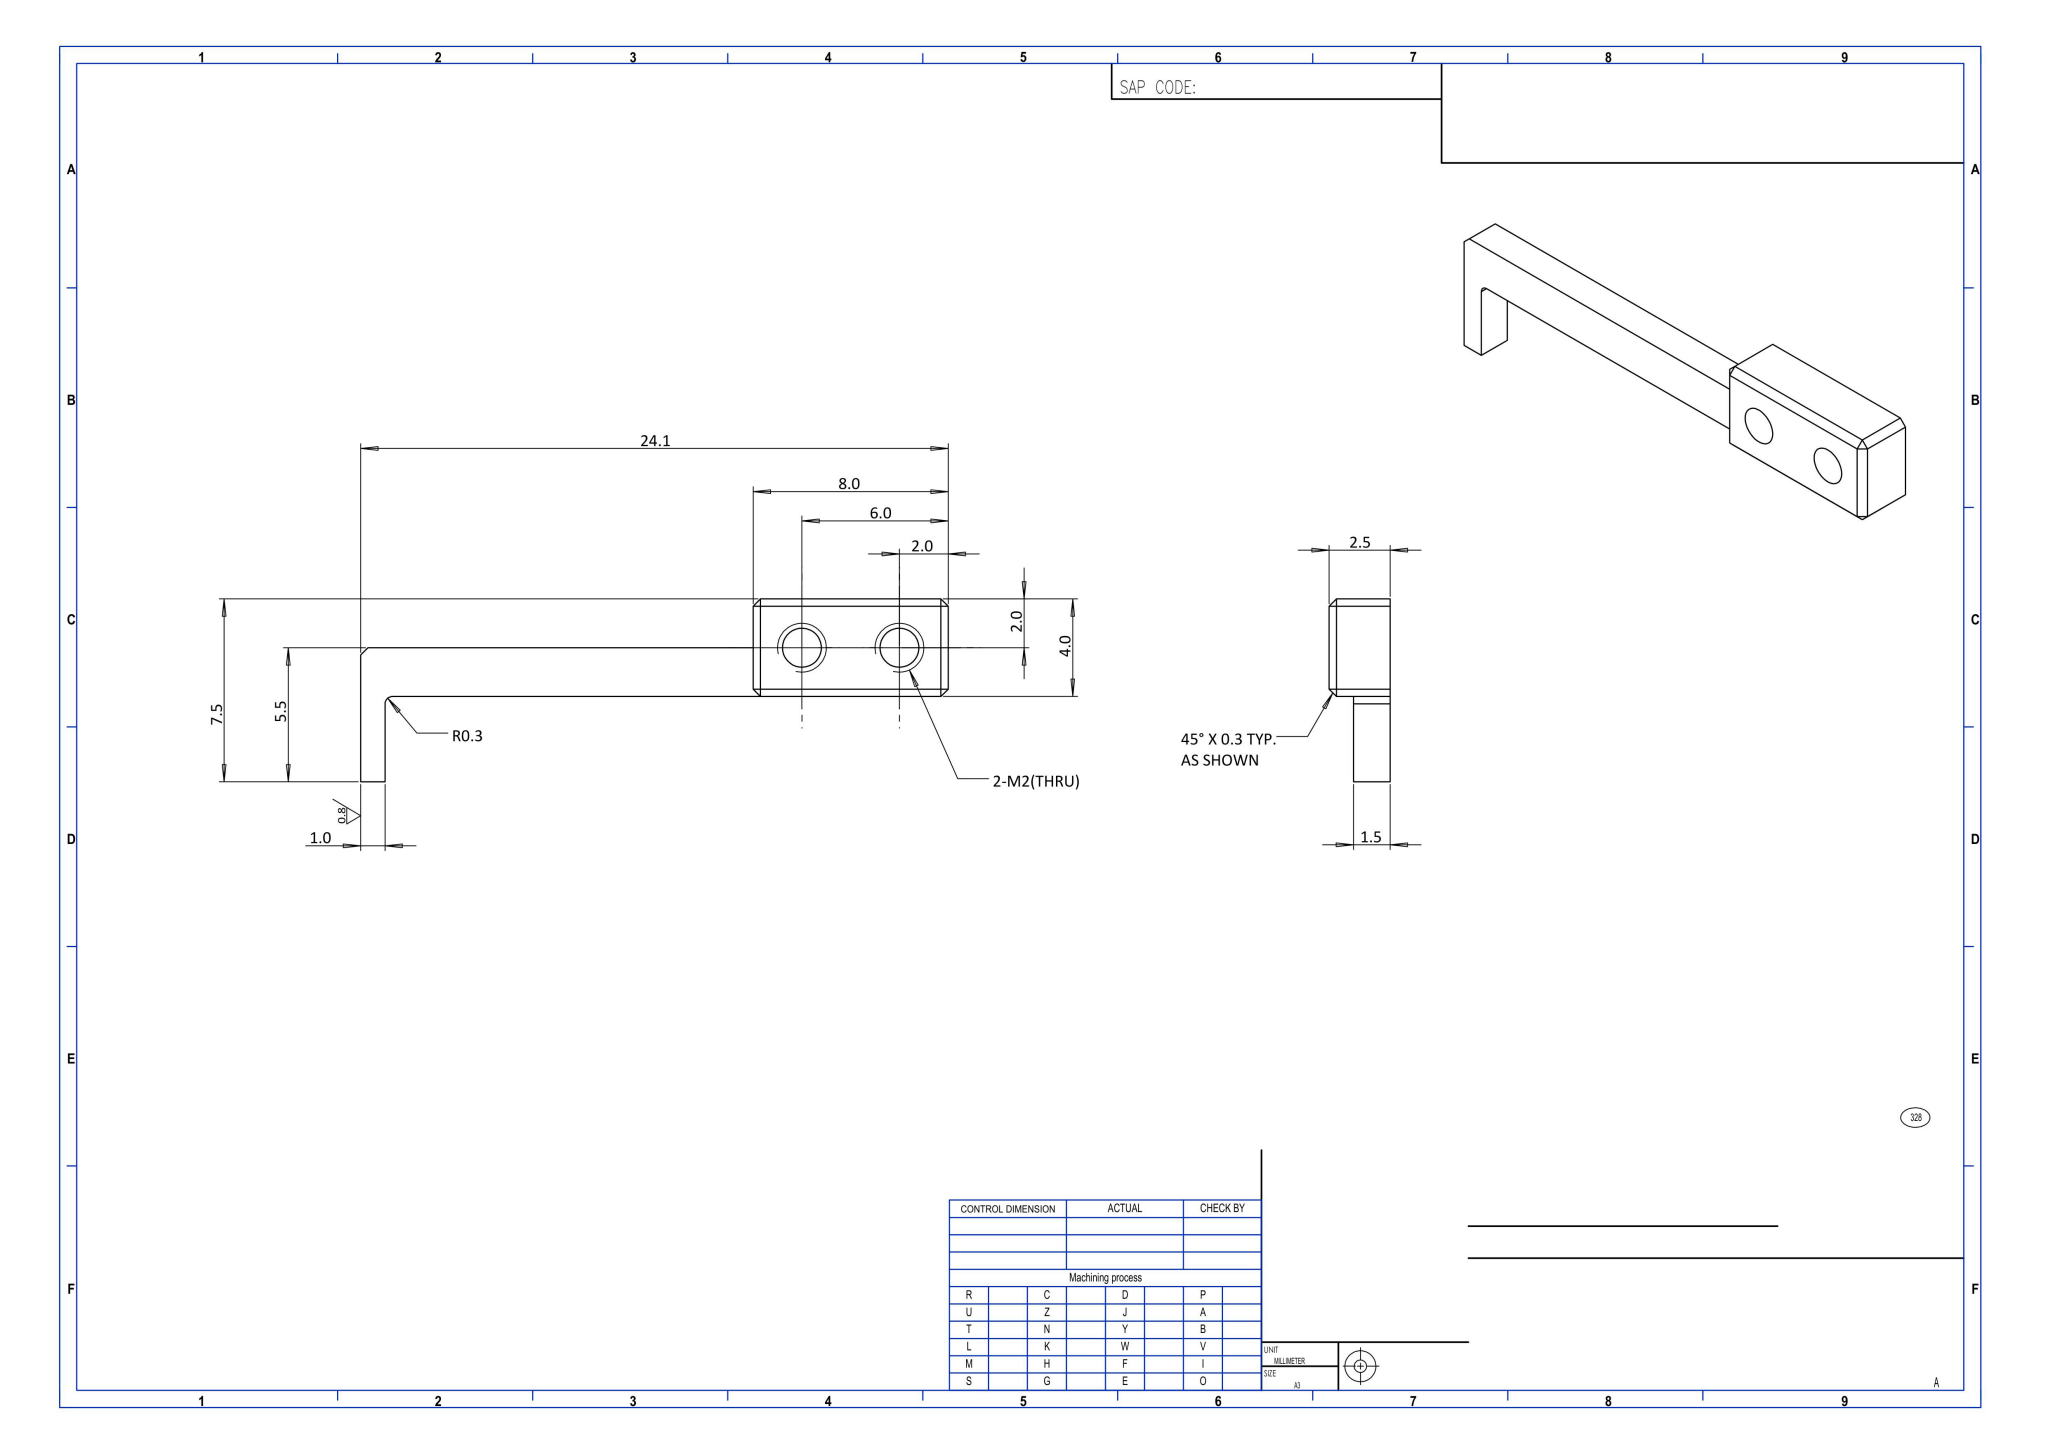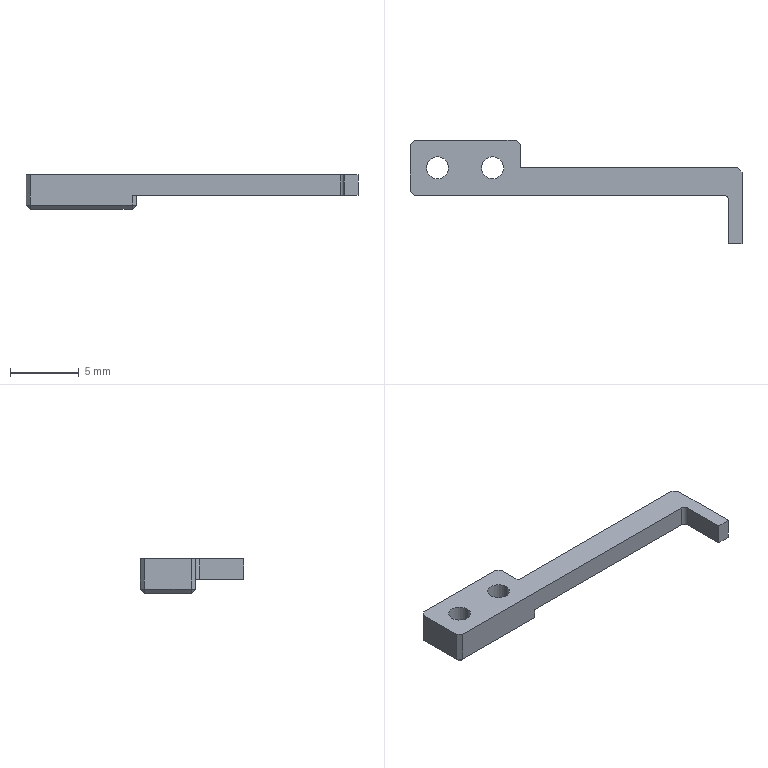Part | NX | mm | 1 solid | 29 faces | box 24.1 x 7.5 x 2.5 mm | volume 122 mm3 | plane 24 | cylinder 5 | commonest cylinder face diameters 1.6 x4 0.6 x1
STEP:
#1=COLOUR_RGB('',0.7529,0.7529,0.7529);
#2=FILL_AREA_STYLE_COLOUR('',#1);
#3=FILL_AREA_STYLE('',(#2));
#4=SURFACE_STYLE_FILL_AREA(#3);
#5=SURFACE_SIDE_STYLE('',(#4));
#6=SURFACE_STYLE_USAGE(.BOTH.,#5);
#7=PRESENTATION_STYLE_ASSIGNMENT((#6));
#8=CARTESIAN_POINT('',(1.2,1.75,-2.5));
#9=VERTEX_POINT('',#8);
#10=CARTESIAN_POINT('',(1.2,1.75,0.));
#11=VERTEX_POINT('',#10);
#12=CARTESIAN_POINT('',(1.2,1.75,0.));
#13=DIRECTION('',(0.,0.,1.));
#14=VECTOR('',#13,1000.);
#15=LINE('',#12,#14);
#16=EDGE_CURVE('',#9,#11,#15,.T.);
#17=ORIENTED_EDGE('',*,*,#16,.F.);
#18=CARTESIAN_POINT('',(2.8,1.75,-2.5));
#19=VERTEX_POINT('',#18);
#20=CARTESIAN_POINT('',(2.,1.75,-2.5));
#21=DIRECTION('',(0.,0.,1.));
#22=DIRECTION('',(1.,0.,0.));
#23=AXIS2_PLACEMENT_3D('',#20,#21,#22);
#24=CIRCLE('',#23,0.8);
#25=EDGE_CURVE('',#19,#9,#24,.T.);
#26=ORIENTED_EDGE('',*,*,#25,.F.);
#27=CARTESIAN_POINT('',(2.8,1.75,0.));
#28=VERTEX_POINT('',#27);
#29=CARTESIAN_POINT('',(2.8,1.75,0.));
#30=DIRECTION('',(0.,0.,1.));
#31=VECTOR('',#30,1000.);
#32=LINE('',#29,#31);
#33=EDGE_CURVE('',#19,#28,#32,.T.);
#34=ORIENTED_EDGE('',*,*,#33,.T.);
#35=CARTESIAN_POINT('',(2.,1.75,0.));
#36=DIRECTION('',(0.,0.,1.));
#37=DIRECTION('',(1.,0.,0.));
#38=AXIS2_PLACEMENT_3D('',#35,#36,#37);
#39=CIRCLE('',#38,0.8);
#40=EDGE_CURVE('',#28,#11,#39,.T.);
#41=ORIENTED_EDGE('',*,*,#40,.T.);
#42=EDGE_LOOP('',(#17,#26,#34,#41));
#43=FACE_OUTER_BOUND('',#42,.T.);
#44=CARTESIAN_POINT('',(2.,1.75,0.));
#45=DIRECTION('',(0.,0.,1.));
#46=DIRECTION('',(1.,0.,0.));
#47=AXIS2_PLACEMENT_3D('',#44,#45,#46);
#48=CYLINDRICAL_SURFACE('',#47,0.8);
#49=ADVANCED_FACE('',(#43),#48,.F.);
#50=STYLED_ITEM('',(#7),#49);
#51=(LENGTH_UNIT()NAMED_UNIT(*)SI_UNIT(.MILLI.,.METRE.));
#52=UNCERTAINTY_MEASURE_WITH_UNIT(LENGTH_MEASURE(0.00001),#51,'','');
#53=(NAMED_UNIT(*)PLANE_ANGLE_UNIT()SI_UNIT($,.RADIAN.));
#54=(NAMED_UNIT(*)SI_UNIT($,.STERADIAN.)SOLID_ANGLE_UNIT());
#55=(GEOMETRIC_REPRESENTATION_CONTEXT(3)GLOBAL_UNCERTAINTY_ASSIGNED_CONTEXT((#52))GLOBAL_UNIT_ASSIGNED_CONTEXT((#51,#53,#54))REPRESENTATION_CONTEXT('',''));
#56=MECHANICAL_DESIGN_GEOMETRIC_PRESENTATION_REPRESENTATION('',(#50),#55);
#57=COLOUR_RGB('',0.7529,0.7529,0.7529);
#58=FILL_AREA_STYLE_COLOUR('',#57);
#59=FILL_AREA_STYLE('',(#58));
#60=SURFACE_STYLE_FILL_AREA(#59);
#61=SURFACE_SIDE_STYLE('',(#60));
#62=SURFACE_STYLE_USAGE(.BOTH.,#61);
#63=PRESENTATION_STYLE_ASSIGNMENT((#62));
#64=CARTESIAN_POINT('',(2.,1.75,-2.5));
#65=DIRECTION('',(0.,0.,1.));
#66=DIRECTION('',(1.,0.,0.));
#67=AXIS2_PLACEMENT_3D('',#64,#65,#66);
#68=CIRCLE('',#67,0.8);
#69=EDGE_CURVE('',#9,#19,#68,.T.);
#70=ORIENTED_EDGE('',*,*,#69,.F.);
#71=ORIENTED_EDGE('',*,*,#16,.T.);
#72=CARTESIAN_POINT('',(2.,1.75,0.));
#73=DIRECTION('',(0.,0.,1.));
#74=DIRECTION('',(1.,0.,0.));
#75=AXIS2_PLACEMENT_3D('',#72,#73,#74);
#76=CIRCLE('',#75,0.8);
#77=EDGE_CURVE('',#11,#28,#76,.T.);
#78=ORIENTED_EDGE('',*,*,#77,.T.);
#79=ORIENTED_EDGE('',*,*,#33,.F.);
#80=EDGE_LOOP('',(#70,#71,#78,#79));
#81=FACE_OUTER_BOUND('',#80,.T.);
#82=CARTESIAN_POINT('',(2.,1.75,0.));
#83=DIRECTION('',(0.,0.,1.));
#84=DIRECTION('',(1.,0.,0.));
#85=AXIS2_PLACEMENT_3D('',#82,#83,#84);
#86=CYLINDRICAL_SURFACE('',#85,0.8);
#87=ADVANCED_FACE('',(#81),#86,.F.);
#88=CARTESIAN_POINT('',(5.2,1.75,-2.5));
#89=VERTEX_POINT('',#88);
#90=CARTESIAN_POINT('',(6.8,1.75,-2.5));
#91=VERTEX_POINT('',#90);
#92=CARTESIAN_POINT('',(6.,1.75,-2.5));
#93=DIRECTION('',(0.,0.,1.));
#94=DIRECTION('',(1.,0.,0.));
#95=AXIS2_PLACEMENT_3D('',#92,#93,#94);
#96=CIRCLE('',#95,0.8);
#97=EDGE_CURVE('',#89,#91,#96,.T.);
#98=ORIENTED_EDGE('',*,*,#97,.F.);
#99=CARTESIAN_POINT('',(5.2,1.75,0.));
#100=VERTEX_POINT('',#99);
#101=CARTESIAN_POINT('',(5.2,1.75,0.));
#102=DIRECTION('',(0.,0.,1.));
#103=VECTOR('',#102,1000.);
#104=LINE('',#101,#103);
#105=EDGE_CURVE('',#89,#100,#104,.T.);
#106=ORIENTED_EDGE('',*,*,#105,.T.);
#107=CARTESIAN_POINT('',(6.8,1.75,0.));
#108=VERTEX_POINT('',#107);
#109=CARTESIAN_POINT('',(6.,1.75,0.));
#110=DIRECTION('',(0.,0.,1.));
#111=DIRECTION('',(1.,0.,0.));
#112=AXIS2_PLACEMENT_3D('',#109,#110,#111);
#113=CIRCLE('',#112,0.8);
#114=EDGE_CURVE('',#100,#108,#113,.T.);
#115=ORIENTED_EDGE('',*,*,#114,.T.);
#116=CARTESIAN_POINT('',(6.8,1.75,0.));
#117=DIRECTION('',(0.,0.,1.));
#118=VECTOR('',#117,1000.);
#119=LINE('',#116,#118);
#120=EDGE_CURVE('',#91,#108,#119,.T.);
#121=ORIENTED_EDGE('',*,*,#120,.F.);
#122=EDGE_LOOP('',(#98,#106,#115,#121));
#123=FACE_OUTER_BOUND('',#122,.T.);
#124=CARTESIAN_POINT('',(6.,1.75,0.));
#125=DIRECTION('',(0.,0.,1.));
#126=DIRECTION('',(1.,0.,0.));
#127=AXIS2_PLACEMENT_3D('',#124,#125,#126);
#128=CYLINDRICAL_SURFACE('',#127,0.8);
#129=ADVANCED_FACE('',(#123),#128,.F.);
#130=CARTESIAN_POINT('',(24.1,-3.75,-1.5));
#131=VERTEX_POINT('',#130);
#132=CARTESIAN_POINT('',(24.1,1.45,-1.5));
#133=VERTEX_POINT('',#132);
#134=CARTESIAN_POINT('',(24.1,-3.75,-1.5));
#135=DIRECTION('',(-0.,1.,0.));
#136=VECTOR('',#135,1000.);
#137=LINE('',#134,#136);
#138=EDGE_CURVE('',#131,#133,#137,.T.);
#139=ORIENTED_EDGE('',*,*,#138,.T.);
#140=CARTESIAN_POINT('',(24.1,1.45,0.));
#141=VERTEX_POINT('',#140);
#142=CARTESIAN_POINT('',(24.1,1.45,0.));
#143=DIRECTION('',(0.,0.,1.));
#144=VECTOR('',#143,1000.);
#145=LINE('',#142,#144);
#146=EDGE_CURVE('',#133,#141,#145,.T.);
#147=ORIENTED_EDGE('',*,*,#146,.T.);
#148=CARTESIAN_POINT('',(24.1,-3.75,0.));
#149=VERTEX_POINT('',#148);
#150=CARTESIAN_POINT('',(24.1,3.75,0.));
#151=DIRECTION('',(0.,1.,0.));
#152=VECTOR('',#151,1000.);
#153=LINE('',#150,#152);
#154=EDGE_CURVE('',#149,#141,#153,.T.);
#155=ORIENTED_EDGE('',*,*,#154,.F.);
#156=CARTESIAN_POINT('',(24.1,-3.75,-2.5));
#157=DIRECTION('',(0.,0.,1.));
#158=VECTOR('',#157,1000.);
#159=LINE('',#156,#158);
#160=EDGE_CURVE('',#131,#149,#159,.T.);
#161=ORIENTED_EDGE('',*,*,#160,.F.);
#162=EDGE_LOOP('',(#139,#147,#155,#161));
#163=FACE_OUTER_BOUND('',#162,.T.);
#164=CARTESIAN_POINT('',(24.1,3.75,-2.5));
#165=DIRECTION('',(1.,0.,0.));
#166=DIRECTION('',(0.,0.,-1.));
#167=AXIS2_PLACEMENT_3D('',#164,#165,#166);
#168=PLANE('',#167);
#169=ADVANCED_FACE('',(#163),#168,.T.);
#170=CARTESIAN_POINT('',(23.1,-3.75,-1.5));
#171=VERTEX_POINT('',#170);
#172=CARTESIAN_POINT('',(24.1,-3.75,-1.5));
#173=DIRECTION('',(1.,0.,-0.));
#174=VECTOR('',#173,1000.);
#175=LINE('',#172,#174);
#176=EDGE_CURVE('',#171,#131,#175,.T.);
#177=ORIENTED_EDGE('',*,*,#176,.T.);
#178=ORIENTED_EDGE('',*,*,#160,.T.);
#179=CARTESIAN_POINT('',(23.1,-3.75,0.));
#180=VERTEX_POINT('',#179);
#181=CARTESIAN_POINT('',(24.1,-3.75,0.));
#182=DIRECTION('',(1.,-0.,0.));
#183=VECTOR('',#182,1000.);
#184=LINE('',#181,#183);
#185=EDGE_CURVE('',#180,#149,#184,.T.);
#186=ORIENTED_EDGE('',*,*,#185,.F.);
#187=CARTESIAN_POINT('',(23.1,-3.75,-2.5));
#188=DIRECTION('',(0.,0.,1.));
#189=VECTOR('',#188,1000.);
#190=LINE('',#187,#189);
#191=EDGE_CURVE('',#171,#180,#190,.T.);
#192=ORIENTED_EDGE('',*,*,#191,.F.);
#193=EDGE_LOOP('',(#177,#178,#186,#192));
#194=FACE_OUTER_BOUND('',#193,.T.);
#195=CARTESIAN_POINT('',(24.1,-3.75,-2.5));
#196=DIRECTION('',(-0.,-1.,0.));
#197=DIRECTION('',(1.,-0.,0.));
#198=AXIS2_PLACEMENT_3D('',#195,#196,#197);
#199=PLANE('',#198);
#200=ADVANCED_FACE('',(#194),#199,.T.);
#201=CARTESIAN_POINT('',(-0.,3.45,0.));
#202=VERTEX_POINT('',#201);
#203=CARTESIAN_POINT('',(-0.,0.05,0.));
#204=VERTEX_POINT('',#203);
#205=CARTESIAN_POINT('',(-0.,3.75,0.));
#206=DIRECTION('',(0.,-1.,0.));
#207=VECTOR('',#206,1000.);
#208=LINE('',#205,#207);
#209=EDGE_CURVE('',#202,#204,#208,.T.);
#210=ORIENTED_EDGE('',*,*,#209,.F.);
#211=CARTESIAN_POINT('',(-0.,3.45,-2.2));
#212=VERTEX_POINT('',#211);
#213=CARTESIAN_POINT('',(-0.,3.45,-2.5));
#214=DIRECTION('',(0.,0.,-1.));
#215=VECTOR('',#214,1000.);
#216=LINE('',#213,#215);
#217=EDGE_CURVE('',#202,#212,#216,.T.);
#218=ORIENTED_EDGE('',*,*,#217,.T.);
#219=CARTESIAN_POINT('',(-0.,0.05,-2.2));
#220=VERTEX_POINT('',#219);
#221=CARTESIAN_POINT('',(-0.,3.75,-2.2));
#222=DIRECTION('',(0.,-1.,0.));
#223=VECTOR('',#222,1000.);
#224=LINE('',#221,#223);
#225=EDGE_CURVE('',#212,#220,#224,.T.);
#226=ORIENTED_EDGE('',*,*,#225,.T.);
#227=CARTESIAN_POINT('',(-0.,0.05,0.));
#228=DIRECTION('',(0.,0.,1.));
#229=VECTOR('',#228,1000.);
#230=LINE('',#227,#229);
#231=EDGE_CURVE('',#220,#204,#230,.T.);
#232=ORIENTED_EDGE('',*,*,#231,.T.);
#233=EDGE_LOOP('',(#210,#218,#226,#232));
#234=FACE_OUTER_BOUND('',#233,.T.);
#235=CARTESIAN_POINT('',(-0.,3.75,-2.5));
#236=DIRECTION('',(-1.,0.,0.));
#237=DIRECTION('',(0.,0.,1.));
#238=AXIS2_PLACEMENT_3D('',#235,#236,#237);
#239=PLANE('',#238);
#240=ADVANCED_FACE('',(#234),#239,.T.);
#241=CARTESIAN_POINT('',(7.7,3.75,-2.2));
#242=VERTEX_POINT('',#241);
#243=CARTESIAN_POINT('',(0.3,3.75,-2.2));
#244=VERTEX_POINT('',#243);
#245=CARTESIAN_POINT('',(24.1,3.75,-2.2));
#246=DIRECTION('',(-1.,-0.,0.));
#247=VECTOR('',#246,1000.);
#248=LINE('',#245,#247);
#249=EDGE_CURVE('',#242,#244,#248,.T.);
#250=ORIENTED_EDGE('',*,*,#249,.T.);
#251=CARTESIAN_POINT('',(0.3,3.75,0.));
#252=VERTEX_POINT('',#251);
#253=CARTESIAN_POINT('',(0.3,3.75,-2.5));
#254=DIRECTION('',(0.,0.,1.));
#255=VECTOR('',#254,1000.);
#256=LINE('',#253,#255);
#257=EDGE_CURVE('',#244,#252,#256,.T.);
#258=ORIENTED_EDGE('',*,*,#257,.T.);
#259=CARTESIAN_POINT('',(7.7,3.75,0.));
#260=VERTEX_POINT('',#259);
#261=CARTESIAN_POINT('',(24.1,3.75,0.));
#262=DIRECTION('',(-1.,-0.,0.));
#263=VECTOR('',#262,1000.);
#264=LINE('',#261,#263);
#265=EDGE_CURVE('',#260,#252,#264,.T.);
#266=ORIENTED_EDGE('',*,*,#265,.F.);
#267=CARTESIAN_POINT('',(7.7,3.75,-2.5));
#268=DIRECTION('',(-0.,-0.,-1.));
#269=VECTOR('',#268,1000.);
#270=LINE('',#267,#269);
#271=EDGE_CURVE('',#260,#242,#270,.T.);
#272=ORIENTED_EDGE('',*,*,#271,.T.);
#273=EDGE_LOOP('',(#250,#258,#266,#272));
#274=FACE_OUTER_BOUND('',#273,.T.);
#275=CARTESIAN_POINT('',(24.1,3.75,-2.5));
#276=DIRECTION('',(-0.,1.,0.));
#277=DIRECTION('',(-1.,-0.,0.));
#278=AXIS2_PLACEMENT_3D('',#275,#276,#277);
#279=PLANE('',#278);
#280=ADVANCED_FACE('',(#274),#279,.T.);
#281=CARTESIAN_POINT('',(0.3,0.05,-2.5));
#282=VERTEX_POINT('',#281);
#283=CARTESIAN_POINT('',(0.3,3.45,-2.5));
#284=VERTEX_POINT('',#283);
#285=CARTESIAN_POINT('',(0.3,0.,-2.5));
#286=DIRECTION('',(0.,1.,0.));
#287=VECTOR('',#286,1000.);
#288=LINE('',#285,#287);
#289=EDGE_CURVE('',#282,#284,#288,.T.);
#290=ORIENTED_EDGE('',*,*,#289,.T.);
#291=CARTESIAN_POINT('',(7.7,3.45,-2.5));
#292=VERTEX_POINT('',#291);
#293=CARTESIAN_POINT('',(-0.,3.45,-2.5));
#294=DIRECTION('',(1.,0.,0.));
#295=VECTOR('',#294,1000.);
#296=LINE('',#293,#295);
#297=EDGE_CURVE('',#284,#292,#296,.T.);
#298=ORIENTED_EDGE('',*,*,#297,.T.);
#299=CARTESIAN_POINT('',(7.7,0.05,-2.5));
#300=VERTEX_POINT('',#299);
#301=CARTESIAN_POINT('',(7.7,-0.25,-2.5));
#302=DIRECTION('',(0.,-1.,0.));
#303=VECTOR('',#302,1000.);
#304=LINE('',#301,#303);
#305=EDGE_CURVE('',#292,#300,#304,.T.);
#306=ORIENTED_EDGE('',*,*,#305,.T.);
#307=CARTESIAN_POINT('',(-0.,0.05,-2.5));
#308=DIRECTION('',(-1.,-0.,0.));
#309=VECTOR('',#308,1000.);
#310=LINE('',#307,#309);
#311=EDGE_CURVE('',#300,#282,#310,.T.);
#312=ORIENTED_EDGE('',*,*,#311,.T.);
#313=EDGE_LOOP('',(#290,#298,#306,#312));
#314=FACE_OUTER_BOUND('',#313,.T.);
#315=ORIENTED_EDGE('',*,*,#25,.T.);
#316=ORIENTED_EDGE('',*,*,#69,.T.);
#317=EDGE_LOOP('',(#315,#316));
#318=FACE_BOUND('',#317,.T.);
#319=CARTESIAN_POINT('',(6.,1.75,-2.5));
#320=DIRECTION('',(0.,0.,1.));
#321=DIRECTION('',(1.,0.,0.));
#322=AXIS2_PLACEMENT_3D('',#319,#320,#321);
#323=CIRCLE('',#322,0.8);
#324=EDGE_CURVE('',#91,#89,#323,.T.);
#325=ORIENTED_EDGE('',*,*,#324,.T.);
#326=ORIENTED_EDGE('',*,*,#97,.T.);
#327=EDGE_LOOP('',(#325,#326));
#328=FACE_BOUND('',#327,.T.);
#329=CARTESIAN_POINT('',(0.,0.,-2.5));
#330=DIRECTION('',(0.,0.,-1.));
#331=DIRECTION('',(-1.,0.,0.));
#332=AXIS2_PLACEMENT_3D('',#329,#330,#331);
#333=PLANE('',#332);
#334=ADVANCED_FACE('',(#314,#318,#328),#333,.T.);
#335=ORIENTED_EDGE('',*,*,#40,.F.);
#336=ORIENTED_EDGE('',*,*,#77,.F.);
#337=EDGE_LOOP('',(#335,#336));
#338=FACE_BOUND('',#337,.T.);
#339=CARTESIAN_POINT('',(6.,1.75,0.));
#340=DIRECTION('',(0.,0.,1.));
#341=DIRECTION('',(1.,0.,0.));
#342=AXIS2_PLACEMENT_3D('',#339,#340,#341);
#343=CIRCLE('',#342,0.8);
#344=EDGE_CURVE('',#108,#100,#343,.T.);
#345=ORIENTED_EDGE('',*,*,#344,.F.);
#346=ORIENTED_EDGE('',*,*,#114,.F.);
#347=EDGE_LOOP('',(#345,#346));
#348=FACE_BOUND('',#347,.T.);
#349=ORIENTED_EDGE('',*,*,#154,.T.);
#350=CARTESIAN_POINT('',(23.8,1.75,0.));
#351=VERTEX_POINT('',#350);
#352=CARTESIAN_POINT('',(24.1,1.45,0.));
#353=DIRECTION('',(-0.7071,0.7071,0.));
#354=VECTOR('',#353,1000.);
#355=LINE('',#352,#354);
#356=EDGE_CURVE('',#141,#351,#355,.T.);
#357=ORIENTED_EDGE('',*,*,#356,.T.);
#358=CARTESIAN_POINT('',(8.,1.75,0.));
#359=VERTEX_POINT('',#358);
#360=CARTESIAN_POINT('',(24.1,1.75,0.));
#361=DIRECTION('',(1.,0.,0.));
#362=VECTOR('',#361,1000.);
#363=LINE('',#360,#362);
#364=EDGE_CURVE('',#359,#351,#363,.T.);
#365=ORIENTED_EDGE('',*,*,#364,.F.);
#366=CARTESIAN_POINT('',(8.,3.45,0.));
#367=VERTEX_POINT('',#366);
#368=CARTESIAN_POINT('',(8.,3.75,0.));
#369=DIRECTION('',(0.,-1.,0.));
#370=VECTOR('',#369,1000.);
#371=LINE('',#368,#370);
#372=EDGE_CURVE('',#367,#359,#371,.T.);
#373=ORIENTED_EDGE('',*,*,#372,.F.);
#374=CARTESIAN_POINT('',(8.,3.45,0.));
#375=DIRECTION('',(-0.7071,0.7071,0.));
#376=VECTOR('',#375,1000.);
#377=LINE('',#374,#376);
#378=EDGE_CURVE('',#367,#260,#377,.T.);
#379=ORIENTED_EDGE('',*,*,#378,.T.);
#380=ORIENTED_EDGE('',*,*,#265,.T.);
#381=CARTESIAN_POINT('',(0.3,3.75,0.));
#382=DIRECTION('',(-0.7071,-0.7071,0.));
#383=VECTOR('',#382,1000.);
#384=LINE('',#381,#383);
#385=EDGE_CURVE('',#252,#202,#384,.T.);
#386=ORIENTED_EDGE('',*,*,#385,.T.);
#387=ORIENTED_EDGE('',*,*,#209,.T.);
#388=CARTESIAN_POINT('',(0.3,-0.25,0.));
#389=VERTEX_POINT('',#388);
#390=CARTESIAN_POINT('',(-0.,0.05,0.));
#391=DIRECTION('',(0.7071,-0.7071,0.));
#392=VECTOR('',#391,1000.);
#393=LINE('',#390,#392);
#394=EDGE_CURVE('',#204,#389,#393,.T.);
#395=ORIENTED_EDGE('',*,*,#394,.T.);
#396=CARTESIAN_POINT('',(22.8,-0.25,0.));
#397=VERTEX_POINT('',#396);
#398=CARTESIAN_POINT('',(23.1,-0.25,0.));
#399=DIRECTION('',(-1.,-0.,0.));
#400=VECTOR('',#399,1000.);
#401=LINE('',#398,#400);
#402=EDGE_CURVE('',#397,#389,#401,.T.);
#403=ORIENTED_EDGE('',*,*,#402,.F.);
#404=CARTESIAN_POINT('',(23.1,-0.55,0.));
#405=VERTEX_POINT('',#404);
#406=CARTESIAN_POINT('',(22.8,-0.55,0.));
#407=DIRECTION('',(0.,0.,-1.));
#408=DIRECTION('',(-1.,0.,0.));
#409=AXIS2_PLACEMENT_3D('',#406,#407,#408);
#410=CIRCLE('',#409,0.3);
#411=EDGE_CURVE('',#397,#405,#410,.T.);
#412=ORIENTED_EDGE('',*,*,#411,.T.);
#413=CARTESIAN_POINT('',(23.1,-0.25,0.));
#414=DIRECTION('',(0.,1.,0.));
#415=VECTOR('',#414,1000.);
#416=LINE('',#413,#415);
#417=EDGE_CURVE('',#180,#405,#416,.T.);
#418=ORIENTED_EDGE('',*,*,#417,.F.);
#419=ORIENTED_EDGE('',*,*,#185,.T.);
#420=EDGE_LOOP('',(#349,#357,#365,#373,#379,#380,#386,#387,#395,#403,#412,#418,#419));
#421=FACE_OUTER_BOUND('',#420,.T.);
#422=CARTESIAN_POINT('',(0.,0.,0.));
#423=DIRECTION('',(0.,0.,-1.));
#424=DIRECTION('',(-1.,0.,0.));
#425=AXIS2_PLACEMENT_3D('',#422,#423,#424);
#426=PLANE('',#425);
#427=ADVANCED_FACE('',(#338,#348,#421),#426,.F.);
#428=ORIENTED_EDGE('',*,*,#105,.F.);
#429=ORIENTED_EDGE('',*,*,#324,.F.);
#430=ORIENTED_EDGE('',*,*,#120,.T.);
#431=ORIENTED_EDGE('',*,*,#344,.T.);
#432=EDGE_LOOP('',(#428,#429,#430,#431));
#433=FACE_OUTER_BOUND('',#432,.T.);
#434=CARTESIAN_POINT('',(6.,1.75,0.));
#435=DIRECTION('',(0.,0.,1.));
#436=DIRECTION('',(1.,0.,0.));
#437=AXIS2_PLACEMENT_3D('',#434,#435,#436);
#438=CYLINDRICAL_SURFACE('',#437,0.8);
#439=ADVANCED_FACE('',(#433),#438,.F.);
#440=ORIENTED_EDGE('',*,*,#417,.T.);
#441=CARTESIAN_POINT('',(23.1,-0.55,-1.5));
#442=VERTEX_POINT('',#441);
#443=CARTESIAN_POINT('',(23.1,-0.55,-1.5));
#444=DIRECTION('',(0.,0.,-1.));
#445=VECTOR('',#444,1000.);
#446=LINE('',#443,#445);
#447=EDGE_CURVE('',#405,#442,#446,.T.);
#448=ORIENTED_EDGE('',*,*,#447,.T.);
#449=CARTESIAN_POINT('',(23.1,-0.25,-1.5));
#450=DIRECTION('',(0.,-1.,0.));
#451=VECTOR('',#450,1000.);
#452=LINE('',#449,#451);
#453=EDGE_CURVE('',#442,#171,#452,.T.);
#454=ORIENTED_EDGE('',*,*,#453,.T.);
#455=ORIENTED_EDGE('',*,*,#191,.T.);
#456=EDGE_LOOP('',(#440,#448,#454,#455));
#457=FACE_OUTER_BOUND('',#456,.T.);
#458=CARTESIAN_POINT('',(23.1,-0.25,-2.5));
#459=DIRECTION('',(1.,0.,0.));
#460=DIRECTION('',(0.,0.,-1.));
#461=AXIS2_PLACEMENT_3D('',#458,#459,#460);
#462=PLANE('',#461);
#463=ADVANCED_FACE('',(#457),#462,.F.);
#464=CARTESIAN_POINT('',(7.7,-0.25,-1.5));
#465=VERTEX_POINT('',#464);
#466=CARTESIAN_POINT('',(22.8,-0.25,-1.5));
#467=VERTEX_POINT('',#466);
#468=CARTESIAN_POINT('',(23.1,-0.25,-1.5));
#469=DIRECTION('',(1.,0.,-0.));
#470=VECTOR('',#469,1000.);
#471=LINE('',#468,#470);
#472=EDGE_CURVE('',#465,#467,#471,.T.);
#473=ORIENTED_EDGE('',*,*,#472,.T.);
#474=CARTESIAN_POINT('',(22.8,-0.25,0.));
#475=DIRECTION('',(0.,0.,1.));
#476=VECTOR('',#475,1000.);
#477=LINE('',#474,#476);
#478=EDGE_CURVE('',#467,#397,#477,.T.);
#479=ORIENTED_EDGE('',*,*,#478,.T.);
#480=ORIENTED_EDGE('',*,*,#402,.T.);
#481=CARTESIAN_POINT('',(0.3,-0.25,-2.2));
#482=VERTEX_POINT('',#481);
#483=CARTESIAN_POINT('',(0.3,-0.25,-2.5));
#484=DIRECTION('',(0.,0.,-1.));
#485=VECTOR('',#484,1000.);
#486=LINE('',#483,#485);
#487=EDGE_CURVE('',#389,#482,#486,.T.);
#488=ORIENTED_EDGE('',*,*,#487,.T.);
#489=CARTESIAN_POINT('',(7.7,-0.25,-2.2));
#490=VERTEX_POINT('',#489);
#491=CARTESIAN_POINT('',(8.,-0.25,-2.2));
#492=DIRECTION('',(1.,0.,0.));
#493=VECTOR('',#492,1000.);
#494=LINE('',#491,#493);
#495=EDGE_CURVE('',#482,#490,#494,.T.);
#496=ORIENTED_EDGE('',*,*,#495,.T.);
#497=CARTESIAN_POINT('',(7.7,-0.25,-2.5));
#498=DIRECTION('',(0.,0.,1.));
#499=VECTOR('',#498,1000.);
#500=LINE('',#497,#499);
#501=EDGE_CURVE('',#490,#465,#500,.T.);
#502=ORIENTED_EDGE('',*,*,#501,.T.);
#503=EDGE_LOOP('',(#473,#479,#480,#488,#496,#502));
#504=FACE_OUTER_BOUND('',#503,.T.);
#505=CARTESIAN_POINT('',(23.1,-0.25,-2.5));
#506=DIRECTION('',(-0.,1.,0.));
#507=DIRECTION('',(-1.,-0.,0.));
#508=AXIS2_PLACEMENT_3D('',#505,#506,#507);
#509=PLANE('',#508);
#510=ADVANCED_FACE('',(#504),#509,.F.);
#511=CARTESIAN_POINT('',(8.,1.75,-1.5));
#512=VERTEX_POINT('',#511);
#513=CARTESIAN_POINT('',(23.8,1.75,-1.5));
#514=VERTEX_POINT('',#513);
#515=CARTESIAN_POINT('',(24.1,1.75,-1.5));
#516=DIRECTION('',(1.,0.,-0.));
#517=VECTOR('',#516,1000.);
#518=LINE('',#515,#517);
#519=EDGE_CURVE('',#512,#514,#518,.T.);
#520=ORIENTED_EDGE('',*,*,#519,.T.);
#521=CARTESIAN_POINT('',(24.1,1.45,-1.5));
#522=DIRECTION('',(0.7071,-0.7071,-0.));
#523=VECTOR('',#522,1000.);
#524=LINE('',#521,#523);
#525=EDGE_CURVE('',#514,#133,#524,.T.);
#526=ORIENTED_EDGE('',*,*,#525,.T.);
#527=ORIENTED_EDGE('',*,*,#138,.F.);
#528=ORIENTED_EDGE('',*,*,#176,.F.);
#529=ORIENTED_EDGE('',*,*,#453,.F.);
#530=CARTESIAN_POINT('',(22.8,-0.55,-1.5));
#531=DIRECTION('',(0.,0.,1.));
#532=DIRECTION('',(1.,0.,0.));
#533=AXIS2_PLACEMENT_3D('',#530,#531,#532);
#534=CIRCLE('',#533,0.3);
#535=EDGE_CURVE('',#442,#467,#534,.T.);
#536=ORIENTED_EDGE('',*,*,#535,.T.);
#537=ORIENTED_EDGE('',*,*,#472,.F.);
#538=CARTESIAN_POINT('',(8.,0.05,-1.5));
#539=VERTEX_POINT('',#538);
#540=CARTESIAN_POINT('',(14.15,6.2,-1.5));
#541=DIRECTION('',(0.7071,0.7071,-0.));
#542=VECTOR('',#541,1000.);
#543=LINE('',#540,#542);
#544=EDGE_CURVE('',#465,#539,#543,.T.);
#545=ORIENTED_EDGE('',*,*,#544,.T.);
#546=CARTESIAN_POINT('',(8.,-3.75,-1.5));
#547=DIRECTION('',(-0.,1.,0.));
#548=VECTOR('',#547,1000.);
#549=LINE('',#546,#548);
#550=EDGE_CURVE('',#539,#512,#549,.T.);
#551=ORIENTED_EDGE('',*,*,#550,.T.);
#552=EDGE_LOOP('',(#520,#526,#527,#528,#529,#536,#537,#545,#551));
#553=FACE_OUTER_BOUND('',#552,.T.);
#554=CARTESIAN_POINT('',(24.1,-3.75,-1.5));
#555=DIRECTION('',(0.,0.,1.));
#556=DIRECTION('',(1.,0.,-0.));
#557=AXIS2_PLACEMENT_3D('',#554,#555,#556);
#558=PLANE('',#557);
#559=ADVANCED_FACE('',(#553),#558,.F.);
#560=ORIENTED_EDGE('',*,*,#550,.F.);
#561=CARTESIAN_POINT('',(8.,0.05,-2.2));
#562=VERTEX_POINT('',#561);
#563=CARTESIAN_POINT('',(8.,0.05,-2.5));
#564=DIRECTION('',(-0.,-0.,-1.));
#565=VECTOR('',#564,1000.);
#566=LINE('',#563,#565);
#567=EDGE_CURVE('',#539,#562,#566,.T.);
#568=ORIENTED_EDGE('',*,*,#567,.T.);
#569=CARTESIAN_POINT('',(8.,3.45,-2.2));
#570=VERTEX_POINT('',#569);
#571=CARTESIAN_POINT('',(8.,3.75,-2.2));
#572=DIRECTION('',(-0.,1.,0.));
#573=VECTOR('',#572,1000.);
#574=LINE('',#571,#573);
#575=EDGE_CURVE('',#562,#570,#574,.T.);
#576=ORIENTED_EDGE('',*,*,#575,.T.);
#577=CARTESIAN_POINT('',(8.,3.45,-0.));
#578=DIRECTION('',(0.,0.,1.));
#579=VECTOR('',#578,1000.);
#580=LINE('',#577,#579);
#581=EDGE_CURVE('',#570,#367,#580,.T.);
#582=ORIENTED_EDGE('',*,*,#581,.T.);
#583=ORIENTED_EDGE('',*,*,#372,.T.);
#584=CARTESIAN_POINT('',(8.,1.75,-2.5));
#585=DIRECTION('',(0.,0.,1.));
#586=VECTOR('',#585,1000.);
#587=LINE('',#584,#586);
#588=EDGE_CURVE('',#512,#359,#587,.T.);
#589=ORIENTED_EDGE('',*,*,#588,.F.);
#590=EDGE_LOOP('',(#560,#568,#576,#582,#583,#589));
#591=FACE_OUTER_BOUND('',#590,.T.);
#592=CARTESIAN_POINT('',(8.,-3.75,-2.5));
#593=DIRECTION('',(-1.,-0.,0.));
#594=DIRECTION('',(0.,0.,1.));
#595=AXIS2_PLACEMENT_3D('',#592,#593,#594);
#596=PLANE('',#595);
#597=ADVANCED_FACE('',(#591),#596,.F.);
#598=ORIENTED_EDGE('',*,*,#364,.T.);
#599=CARTESIAN_POINT('',(23.8,1.75,-1.5));
#600=DIRECTION('',(0.,0.,-1.));
#601=VECTOR('',#600,1000.);
#602=LINE('',#599,#601);
#603=EDGE_CURVE('',#351,#514,#602,.T.);
#604=ORIENTED_EDGE('',*,*,#603,.T.);
#605=ORIENTED_EDGE('',*,*,#519,.F.);
#606=ORIENTED_EDGE('',*,*,#588,.T.);
#607=EDGE_LOOP('',(#598,#604,#605,#606));
#608=FACE_OUTER_BOUND('',#607,.T.);
#609=CARTESIAN_POINT('',(24.1,1.75,-2.5));
#610=DIRECTION('',(0.,-1.,0.));
#611=DIRECTION('',(1.,0.,0.));
#612=AXIS2_PLACEMENT_3D('',#609,#610,#611);
#613=PLANE('',#612);
#614=ADVANCED_FACE('',(#608),#613,.F.);
#615=ORIENTED_EDGE('',*,*,#525,.F.);
#616=ORIENTED_EDGE('',*,*,#603,.F.);
#617=ORIENTED_EDGE('',*,*,#356,.F.);
#618=ORIENTED_EDGE('',*,*,#146,.F.);
#619=EDGE_LOOP('',(#615,#616,#617,#618));
#620=FACE_OUTER_BOUND('',#619,.T.);
#621=CARTESIAN_POINT('',(24.1,1.45,-2.5));
#622=DIRECTION('',(0.7071,0.7071,0.));
#623=DIRECTION('',(0.,0.,-1.));
#624=AXIS2_PLACEMENT_3D('',#621,#622,#623);
#625=PLANE('',#624);
#626=ADVANCED_FACE('',(#620),#625,.T.);
#627=ORIENTED_EDGE('',*,*,#544,.F.);
#628=ORIENTED_EDGE('',*,*,#501,.F.);
#629=CARTESIAN_POINT('',(7.7,-0.25,-2.2));
#630=DIRECTION('',(-0.7071,-0.7071,-0.));
#631=VECTOR('',#630,1000.);
#632=LINE('',#629,#631);
#633=EDGE_CURVE('',#562,#490,#632,.T.);
#634=ORIENTED_EDGE('',*,*,#633,.F.);
#635=ORIENTED_EDGE('',*,*,#567,.F.);
#636=EDGE_LOOP('',(#627,#628,#634,#635));
#637=FACE_OUTER_BOUND('',#636,.T.);
#638=CARTESIAN_POINT('',(7.7,-0.25,-2.5));
#639=DIRECTION('',(-0.7071,0.7071,0.));
#640=DIRECTION('',(0.,0.,1.));
#641=AXIS2_PLACEMENT_3D('',#638,#639,#640);
#642=PLANE('',#641);
#643=ADVANCED_FACE('',(#637),#642,.F.);
#644=ORIENTED_EDGE('',*,*,#394,.F.);
#645=ORIENTED_EDGE('',*,*,#231,.F.);
#646=CARTESIAN_POINT('',(-0.,0.05,-2.2));
#647=DIRECTION('',(-0.7071,0.7071,0.));
#648=VECTOR('',#647,1000.);
#649=LINE('',#646,#648);
#650=EDGE_CURVE('',#482,#220,#649,.T.);
#651=ORIENTED_EDGE('',*,*,#650,.F.);
#652=ORIENTED_EDGE('',*,*,#487,.F.);
#653=EDGE_LOOP('',(#644,#645,#651,#652));
#654=FACE_OUTER_BOUND('',#653,.T.);
#655=CARTESIAN_POINT('',(-0.,0.05,-2.5));
#656=DIRECTION('',(-0.7071,-0.7071,0.));
#657=DIRECTION('',(0.,0.,-1.));
#658=AXIS2_PLACEMENT_3D('',#655,#656,#657);
#659=PLANE('',#658);
#660=ADVANCED_FACE('',(#654),#659,.T.);
#661=CARTESIAN_POINT('',(7.7,-0.25,-2.2));
#662=DIRECTION('',(-0.,0.7071,-0.7071));
#663=VECTOR('',#662,1000.);
#664=LINE('',#661,#663);
#665=EDGE_CURVE('',#490,#300,#664,.T.);
#666=ORIENTED_EDGE('',*,*,#665,.F.);
#667=ORIENTED_EDGE('',*,*,#495,.F.);
#668=CARTESIAN_POINT('',(0.3,-0.1,-2.35));
#669=DIRECTION('',(-0.,-0.7071,0.7071));
#670=VECTOR('',#669,1000.);
#671=LINE('',#668,#670);
#672=EDGE_CURVE('',#282,#482,#671,.T.);
#673=ORIENTED_EDGE('',*,*,#672,.F.);
#674=ORIENTED_EDGE('',*,*,#311,.F.);
#675=EDGE_LOOP('',(#666,#667,#673,#674));
#676=FACE_OUTER_BOUND('',#675,.T.);
#677=CARTESIAN_POINT('',(-0.,0.05,-2.5));
#678=DIRECTION('',(0.,-0.7071,-0.7071));
#679=DIRECTION('',(1.,0.,0.));
#680=AXIS2_PLACEMENT_3D('',#677,#678,#679);
#681=PLANE('',#680);
#682=ADVANCED_FACE('',(#676),#681,.T.);
#683=ORIENTED_EDGE('',*,*,#633,.T.);
#684=ORIENTED_EDGE('',*,*,#665,.T.);
#685=CARTESIAN_POINT('',(7.85,0.05,-2.35));
#686=DIRECTION('',(-0.7071,0.,-0.7071));
#687=VECTOR('',#686,1000.);
#688=LINE('',#685,#687);
#689=EDGE_CURVE('',#562,#300,#688,.T.);
#690=ORIENTED_EDGE('',*,*,#689,.F.);
#691=EDGE_LOOP('',(#683,#684,#690));
#692=FACE_OUTER_BOUND('',#691,.T.);
#693=CARTESIAN_POINT('',(7.7,-0.25,-2.2));
#694=DIRECTION('',(0.5774,-0.5774,-0.5774));
#695=DIRECTION('',(-0.7071,0.,-0.7071));
#696=AXIS2_PLACEMENT_3D('',#693,#694,#695);
#697=PLANE('',#696);
#698=ADVANCED_FACE('',(#692),#697,.T.);
#699=ORIENTED_EDGE('',*,*,#672,.T.);
#700=ORIENTED_EDGE('',*,*,#650,.T.);
#701=CARTESIAN_POINT('',(-0.,0.05,-2.2));
#702=DIRECTION('',(-0.7071,0.,0.7071));
#703=VECTOR('',#702,1000.);
#704=LINE('',#701,#703);
#705=EDGE_CURVE('',#282,#220,#704,.T.);
#706=ORIENTED_EDGE('',*,*,#705,.F.);
#707=EDGE_LOOP('',(#699,#700,#706));
#708=FACE_OUTER_BOUND('',#707,.T.);
#709=CARTESIAN_POINT('',(-0.,0.05,-2.2));
#710=DIRECTION('',(-0.5774,-0.5774,-0.5774));
#711=DIRECTION('',(-0.7071,0.,0.7071));
#712=AXIS2_PLACEMENT_3D('',#709,#710,#711);
#713=PLANE('',#712);
#714=ADVANCED_FACE('',(#708),#713,.T.);
#715=ORIENTED_EDGE('',*,*,#689,.T.);
#716=ORIENTED_EDGE('',*,*,#305,.F.);
#717=CARTESIAN_POINT('',(7.7,3.45,-2.5));
#718=DIRECTION('',(-0.7071,-0.,-0.7071));
#719=VECTOR('',#718,1000.);
#720=LINE('',#717,#719);
#721=EDGE_CURVE('',#570,#292,#720,.T.);
#722=ORIENTED_EDGE('',*,*,#721,.F.);
#723=ORIENTED_EDGE('',*,*,#575,.F.);
#724=EDGE_LOOP('',(#715,#716,#722,#723));
#725=FACE_OUTER_BOUND('',#724,.T.);
#726=CARTESIAN_POINT('',(8.,-3.75,-2.2));
#727=DIRECTION('',(0.7071,0.,-0.7071));
#728=DIRECTION('',(0.,-1.,0.));
#729=AXIS2_PLACEMENT_3D('',#726,#727,#728);
#730=PLANE('',#729);
#731=ADVANCED_FACE('',(#725),#730,.T.);
#732=ORIENTED_EDGE('',*,*,#378,.F.);
#733=ORIENTED_EDGE('',*,*,#581,.F.);
#734=CARTESIAN_POINT('',(7.85,3.6,-2.2));
#735=DIRECTION('',(0.7071,-0.7071,0.));
#736=VECTOR('',#735,1000.);
#737=LINE('',#734,#736);
#738=EDGE_CURVE('',#242,#570,#737,.T.);
#739=ORIENTED_EDGE('',*,*,#738,.F.);
#740=ORIENTED_EDGE('',*,*,#271,.F.);
#741=EDGE_LOOP('',(#732,#733,#739,#740));
#742=FACE_OUTER_BOUND('',#741,.T.);
#743=CARTESIAN_POINT('',(8.,3.45,-2.5));
#744=DIRECTION('',(0.7071,0.7071,-0.));
#745=DIRECTION('',(-0.,-0.,-1.));
#746=AXIS2_PLACEMENT_3D('',#743,#744,#745);
#747=PLANE('',#746);
#748=ADVANCED_FACE('',(#742),#747,.T.);
#749=ORIENTED_EDGE('',*,*,#385,.F.);
#750=ORIENTED_EDGE('',*,*,#257,.F.);
#751=CARTESIAN_POINT('',(0.3,3.75,-2.2));
#752=DIRECTION('',(0.7071,0.7071,-0.));
#753=VECTOR('',#752,1000.);
#754=LINE('',#751,#753);
#755=EDGE_CURVE('',#212,#244,#754,.T.);
#756=ORIENTED_EDGE('',*,*,#755,.F.);
#757=ORIENTED_EDGE('',*,*,#217,.F.);
#758=EDGE_LOOP('',(#749,#750,#756,#757));
#759=FACE_OUTER_BOUND('',#758,.T.);
#760=CARTESIAN_POINT('',(0.3,3.75,-2.5));
#761=DIRECTION('',(0.7071,-0.7071,0.));
#762=DIRECTION('',(0.,0.,1.));
#763=AXIS2_PLACEMENT_3D('',#760,#761,#762);
#764=PLANE('',#763);
#765=ADVANCED_FACE('',(#759),#764,.F.);
#766=ORIENTED_EDGE('',*,*,#705,.T.);
#767=ORIENTED_EDGE('',*,*,#225,.F.);
#768=CARTESIAN_POINT('',(0.15,3.45,-2.35));
#769=DIRECTION('',(-0.7071,-0.,0.7071));
#770=VECTOR('',#769,1000.);
#771=LINE('',#768,#770);
#772=EDGE_CURVE('',#284,#212,#771,.T.);
#773=ORIENTED_EDGE('',*,*,#772,.F.);
#774=ORIENTED_EDGE('',*,*,#289,.F.);
#775=EDGE_LOOP('',(#766,#767,#773,#774));
#776=FACE_OUTER_BOUND('',#775,.T.);
#777=CARTESIAN_POINT('',(-0.,3.75,-2.2));
#778=DIRECTION('',(0.7071,0.,0.7071));
#779=DIRECTION('',(0.,-1.,0.));
#780=AXIS2_PLACEMENT_3D('',#777,#778,#779);
#781=PLANE('',#780);
#782=ADVANCED_FACE('',(#776),#781,.F.);
#783=ORIENTED_EDGE('',*,*,#738,.T.);
#784=ORIENTED_EDGE('',*,*,#721,.T.);
#785=CARTESIAN_POINT('',(7.7,3.45,-2.5));
#786=DIRECTION('',(-0.,-0.7071,-0.7071));
#787=VECTOR('',#786,1000.);
#788=LINE('',#785,#787);
#789=EDGE_CURVE('',#242,#292,#788,.T.);
#790=ORIENTED_EDGE('',*,*,#789,.F.);
#791=EDGE_LOOP('',(#783,#784,#790));
#792=FACE_OUTER_BOUND('',#791,.T.);
#793=CARTESIAN_POINT('',(7.7,3.45,-2.5));
#794=DIRECTION('',(0.5774,0.5774,-0.5774));
#795=DIRECTION('',(-0.7071,0.,-0.7071));
#796=AXIS2_PLACEMENT_3D('',#793,#794,#795);
#797=PLANE('',#796);
#798=ADVANCED_FACE('',(#792),#797,.T.);
#799=ORIENTED_EDGE('',*,*,#772,.T.);
#800=ORIENTED_EDGE('',*,*,#755,.T.);
#801=CARTESIAN_POINT('',(0.3,3.75,-2.2));
#802=DIRECTION('',(-0.,0.7071,0.7071));
#803=VECTOR('',#802,1000.);
#804=LINE('',#801,#803);
#805=EDGE_CURVE('',#284,#244,#804,.T.);
#806=ORIENTED_EDGE('',*,*,#805,.F.);
#807=EDGE_LOOP('',(#799,#800,#806));
#808=FACE_OUTER_BOUND('',#807,.T.);
#809=CARTESIAN_POINT('',(0.3,3.75,-2.2));
#810=DIRECTION('',(-0.5774,0.5774,-0.5774));
#811=DIRECTION('',(-0.7071,0.,0.7071));
#812=AXIS2_PLACEMENT_3D('',#809,#810,#811);
#813=PLANE('',#812);
#814=ADVANCED_FACE('',(#808),#813,.T.);
#815=ORIENTED_EDGE('',*,*,#789,.T.);
#816=ORIENTED_EDGE('',*,*,#297,.F.);
#817=ORIENTED_EDGE('',*,*,#805,.T.);
#818=ORIENTED_EDGE('',*,*,#249,.F.);
#819=EDGE_LOOP('',(#815,#816,#817,#818));
#820=FACE_OUTER_BOUND('',#819,.T.);
#821=CARTESIAN_POINT('',(24.1,3.75,-2.2));
#822=DIRECTION('',(0.,-0.7071,0.7071));
#823=DIRECTION('',(-1.,-0.,0.));
#824=AXIS2_PLACEMENT_3D('',#821,#822,#823);
#825=PLANE('',#824);
#826=ADVANCED_FACE('',(#820),#825,.F.);
#827=ORIENTED_EDGE('',*,*,#535,.F.);
#828=ORIENTED_EDGE('',*,*,#447,.F.);
#829=ORIENTED_EDGE('',*,*,#411,.F.);
#830=ORIENTED_EDGE('',*,*,#478,.F.);
#831=EDGE_LOOP('',(#827,#828,#829,#830));
#832=FACE_OUTER_BOUND('',#831,.T.);
#833=CARTESIAN_POINT('',(22.8,-0.55,-2.5));
#834=DIRECTION('',(0.,0.,-1.));
#835=DIRECTION('',(-1.,0.,0.));
#836=AXIS2_PLACEMENT_3D('',#833,#834,#835);
#837=CYLINDRICAL_SURFACE('',#836,0.3);
#838=ADVANCED_FACE('',(#832),#837,.F.);
#839=CLOSED_SHELL('',(#87,#129,#169,#200,#240,#280,#334,#427,#439,#49,#463,#510,#559,#597,#614,#626,#643,#660,#682,#698,#714,#731,#748,#765,#782,#798,#814,#826,#838));
#840=MANIFOLD_SOLID_BREP('',#839);
#841=STYLED_ITEM('',(#63),#840);
#842=PRESENTATION_LAYER_ASSIGNMENT('','',(#841));
#843=COLOUR_RGB('',0.7529,0.7529,0.7529);
#844=FILL_AREA_STYLE_COLOUR('',#843);
#845=FILL_AREA_STYLE('',(#844));
#846=SURFACE_STYLE_FILL_AREA(#845);
#847=SURFACE_SIDE_STYLE('',(#846));
#848=SURFACE_STYLE_USAGE(.BOTH.,#847);
#849=PRESENTATION_STYLE_ASSIGNMENT((#848));
#850=CARTESIAN_POINT('',(0.,0.,0.));
#851=DIRECTION('',(0.,0.,1.));
#852=DIRECTION('',(1.,0.,0.));
#853=AXIS2_PLACEMENT_3D('',#850,#851,#852);
#854=(LENGTH_UNIT()NAMED_UNIT(*)SI_UNIT(.MILLI.,.METRE.));
#855=UNCERTAINTY_MEASURE_WITH_UNIT(LENGTH_MEASURE(0.00001),#854,'','');
#856=(NAMED_UNIT(*)PLANE_ANGLE_UNIT()SI_UNIT($,.RADIAN.));
#857=(NAMED_UNIT(*)SI_UNIT($,.STERADIAN.)SOLID_ANGLE_UNIT());
#858=(GEOMETRIC_REPRESENTATION_CONTEXT(3)GLOBAL_UNCERTAINTY_ASSIGNED_CONTEXT((#855))GLOBAL_UNIT_ASSIGNED_CONTEXT((#854,#856,#857))REPRESENTATION_CONTEXT('',''));
#859=ADVANCED_BREP_SHAPE_REPRESENTATION('',(#840,#853),#858);
#860=STYLED_ITEM('',(#849),#859);
#861=(LENGTH_UNIT()NAMED_UNIT(*)SI_UNIT(.MILLI.,.METRE.));
#862=UNCERTAINTY_MEASURE_WITH_UNIT(LENGTH_MEASURE(0.00001),#861,'','');
#863=(NAMED_UNIT(*)PLANE_ANGLE_UNIT()SI_UNIT($,.RADIAN.));
#864=(NAMED_UNIT(*)SI_UNIT($,.STERADIAN.)SOLID_ANGLE_UNIT());
#865=(GEOMETRIC_REPRESENTATION_CONTEXT(3)GLOBAL_UNCERTAINTY_ASSIGNED_CONTEXT((#862))GLOBAL_UNIT_ASSIGNED_CONTEXT((#861,#863,#864))REPRESENTATION_CONTEXT('',''));
#866=MECHANICAL_DESIGN_GEOMETRIC_PRESENTATION_REPRESENTATION('',(#860),#865);
#867=COLOUR_RGB('',0.7529,0.7529,0.7529);
#868=FILL_AREA_STYLE_COLOUR('',#867);
#869=FILL_AREA_STYLE('',(#868));
#870=SURFACE_STYLE_FILL_AREA(#869);
#871=SURFACE_SIDE_STYLE('',(#870));
#872=SURFACE_STYLE_USAGE(.BOTH.,#871);
#873=PRESENTATION_STYLE_ASSIGNMENT((#872));
#874=STYLED_ITEM('',(#873),#129);
#875=(LENGTH_UNIT()NAMED_UNIT(*)SI_UNIT(.MILLI.,.METRE.));
#876=UNCERTAINTY_MEASURE_WITH_UNIT(LENGTH_MEASURE(0.00001),#875,'','');
#877=(NAMED_UNIT(*)PLANE_ANGLE_UNIT()SI_UNIT($,.RADIAN.));
#878=(NAMED_UNIT(*)SI_UNIT($,.STERADIAN.)SOLID_ANGLE_UNIT());
#879=(GEOMETRIC_REPRESENTATION_CONTEXT(3)GLOBAL_UNCERTAINTY_ASSIGNED_CONTEXT((#876))GLOBAL_UNIT_ASSIGNED_CONTEXT((#875,#877,#878))REPRESENTATION_CONTEXT('',''));
#880=MECHANICAL_DESIGN_GEOMETRIC_PRESENTATION_REPRESENTATION('',(#874),#879);
#881=COLOUR_RGB('',0.7529,0.7529,0.7529);
#882=FILL_AREA_STYLE_COLOUR('',#881);
#883=FILL_AREA_STYLE('',(#882));
#884=SURFACE_STYLE_FILL_AREA(#883);
#885=SURFACE_SIDE_STYLE('',(#884));
#886=SURFACE_STYLE_USAGE(.BOTH.,#885);
#887=PRESENTATION_STYLE_ASSIGNMENT((#886));
#888=STYLED_ITEM('',(#887),#87);
#889=PRESENTATION_LAYER_ASSIGNMENT('','',(#888));
#890=COLOUR_RGB('',0.7529,0.7529,0.7529);
#891=FILL_AREA_STYLE_COLOUR('',#890);
#892=FILL_AREA_STYLE('',(#891));
#893=SURFACE_STYLE_FILL_AREA(#892);
#894=SURFACE_SIDE_STYLE('',(#893));
#895=SURFACE_STYLE_USAGE(.BOTH.,#894);
#896=PRESENTATION_STYLE_ASSIGNMENT((#895));
#897=STYLED_ITEM('',(#896),#439);
#898=(LENGTH_UNIT()NAMED_UNIT(*)SI_UNIT(.MILLI.,.METRE.));
#899=UNCERTAINTY_MEASURE_WITH_UNIT(LENGTH_MEASURE(0.00001),#898,'','');
#900=(NAMED_UNIT(*)PLANE_ANGLE_UNIT()SI_UNIT($,.RADIAN.));
#901=(NAMED_UNIT(*)SI_UNIT($,.STERADIAN.)SOLID_ANGLE_UNIT());
#902=(GEOMETRIC_REPRESENTATION_CONTEXT(3)GLOBAL_UNCERTAINTY_ASSIGNED_CONTEXT((#899))GLOBAL_UNIT_ASSIGNED_CONTEXT((#898,#900,#901))REPRESENTATION_CONTEXT('',''));
#903=MECHANICAL_DESIGN_GEOMETRIC_PRESENTATION_REPRESENTATION('',(#897),#902);
#904=PRESENTATION_LAYER_ASSIGNMENT('','',(#50));
#905=PRESENTATION_LAYER_ASSIGNMENT('','',(#860));
#906=PRESENTATION_LAYER_ASSIGNMENT('','',(#874));
#907=(LENGTH_UNIT()NAMED_UNIT(*)SI_UNIT(.MILLI.,.METRE.));
#908=UNCERTAINTY_MEASURE_WITH_UNIT(LENGTH_MEASURE(0.00001),#907,'','');
#909=(NAMED_UNIT(*)PLANE_ANGLE_UNIT()SI_UNIT($,.RADIAN.));
#910=(NAMED_UNIT(*)SI_UNIT($,.STERADIAN.)SOLID_ANGLE_UNIT());
#911=(GEOMETRIC_REPRESENTATION_CONTEXT(3)GLOBAL_UNCERTAINTY_ASSIGNED_CONTEXT((#908))GLOBAL_UNIT_ASSIGNED_CONTEXT((#907,#909,#910))REPRESENTATION_CONTEXT('',''));
#912=MECHANICAL_DESIGN_GEOMETRIC_PRESENTATION_REPRESENTATION('',(#841),#911);
#913=(LENGTH_UNIT()NAMED_UNIT(*)SI_UNIT(.MILLI.,.METRE.));
#914=UNCERTAINTY_MEASURE_WITH_UNIT(LENGTH_MEASURE(0.00001),#913,'','');
#915=(NAMED_UNIT(*)PLANE_ANGLE_UNIT()SI_UNIT($,.RADIAN.));
#916=(NAMED_UNIT(*)SI_UNIT($,.STERADIAN.)SOLID_ANGLE_UNIT());
#917=(GEOMETRIC_REPRESENTATION_CONTEXT(3)GLOBAL_UNCERTAINTY_ASSIGNED_CONTEXT((#914))GLOBAL_UNIT_ASSIGNED_CONTEXT((#913,#915,#916))REPRESENTATION_CONTEXT('',''));
#918=MECHANICAL_DESIGN_GEOMETRIC_PRESENTATION_REPRESENTATION('',(#888),#917);
#919=PRESENTATION_LAYER_ASSIGNMENT('','',(#897));